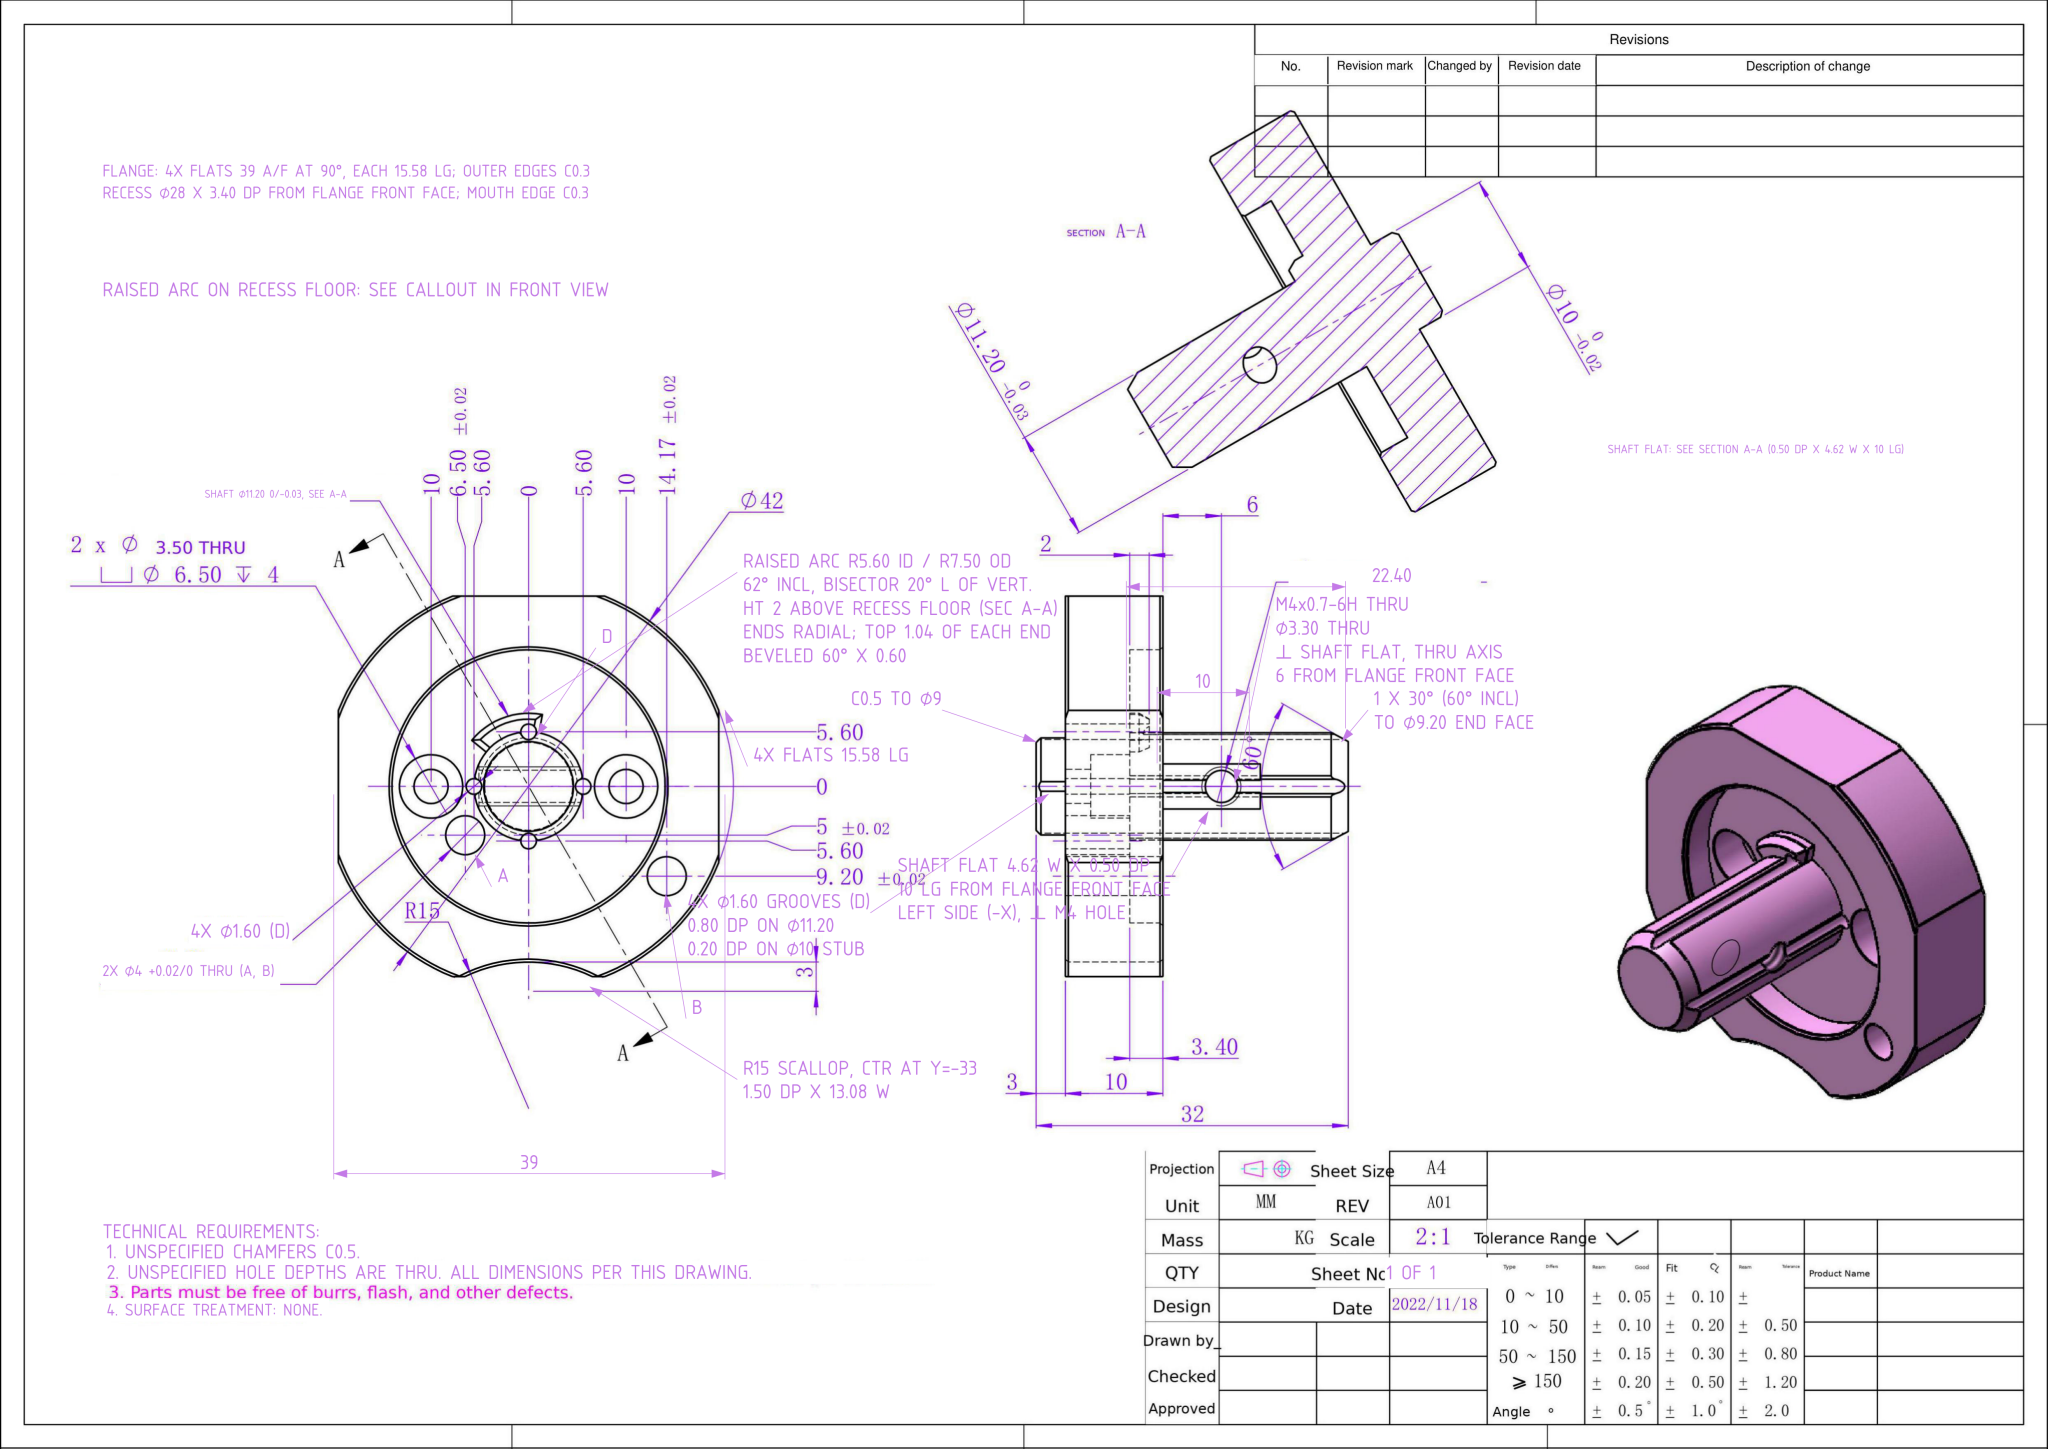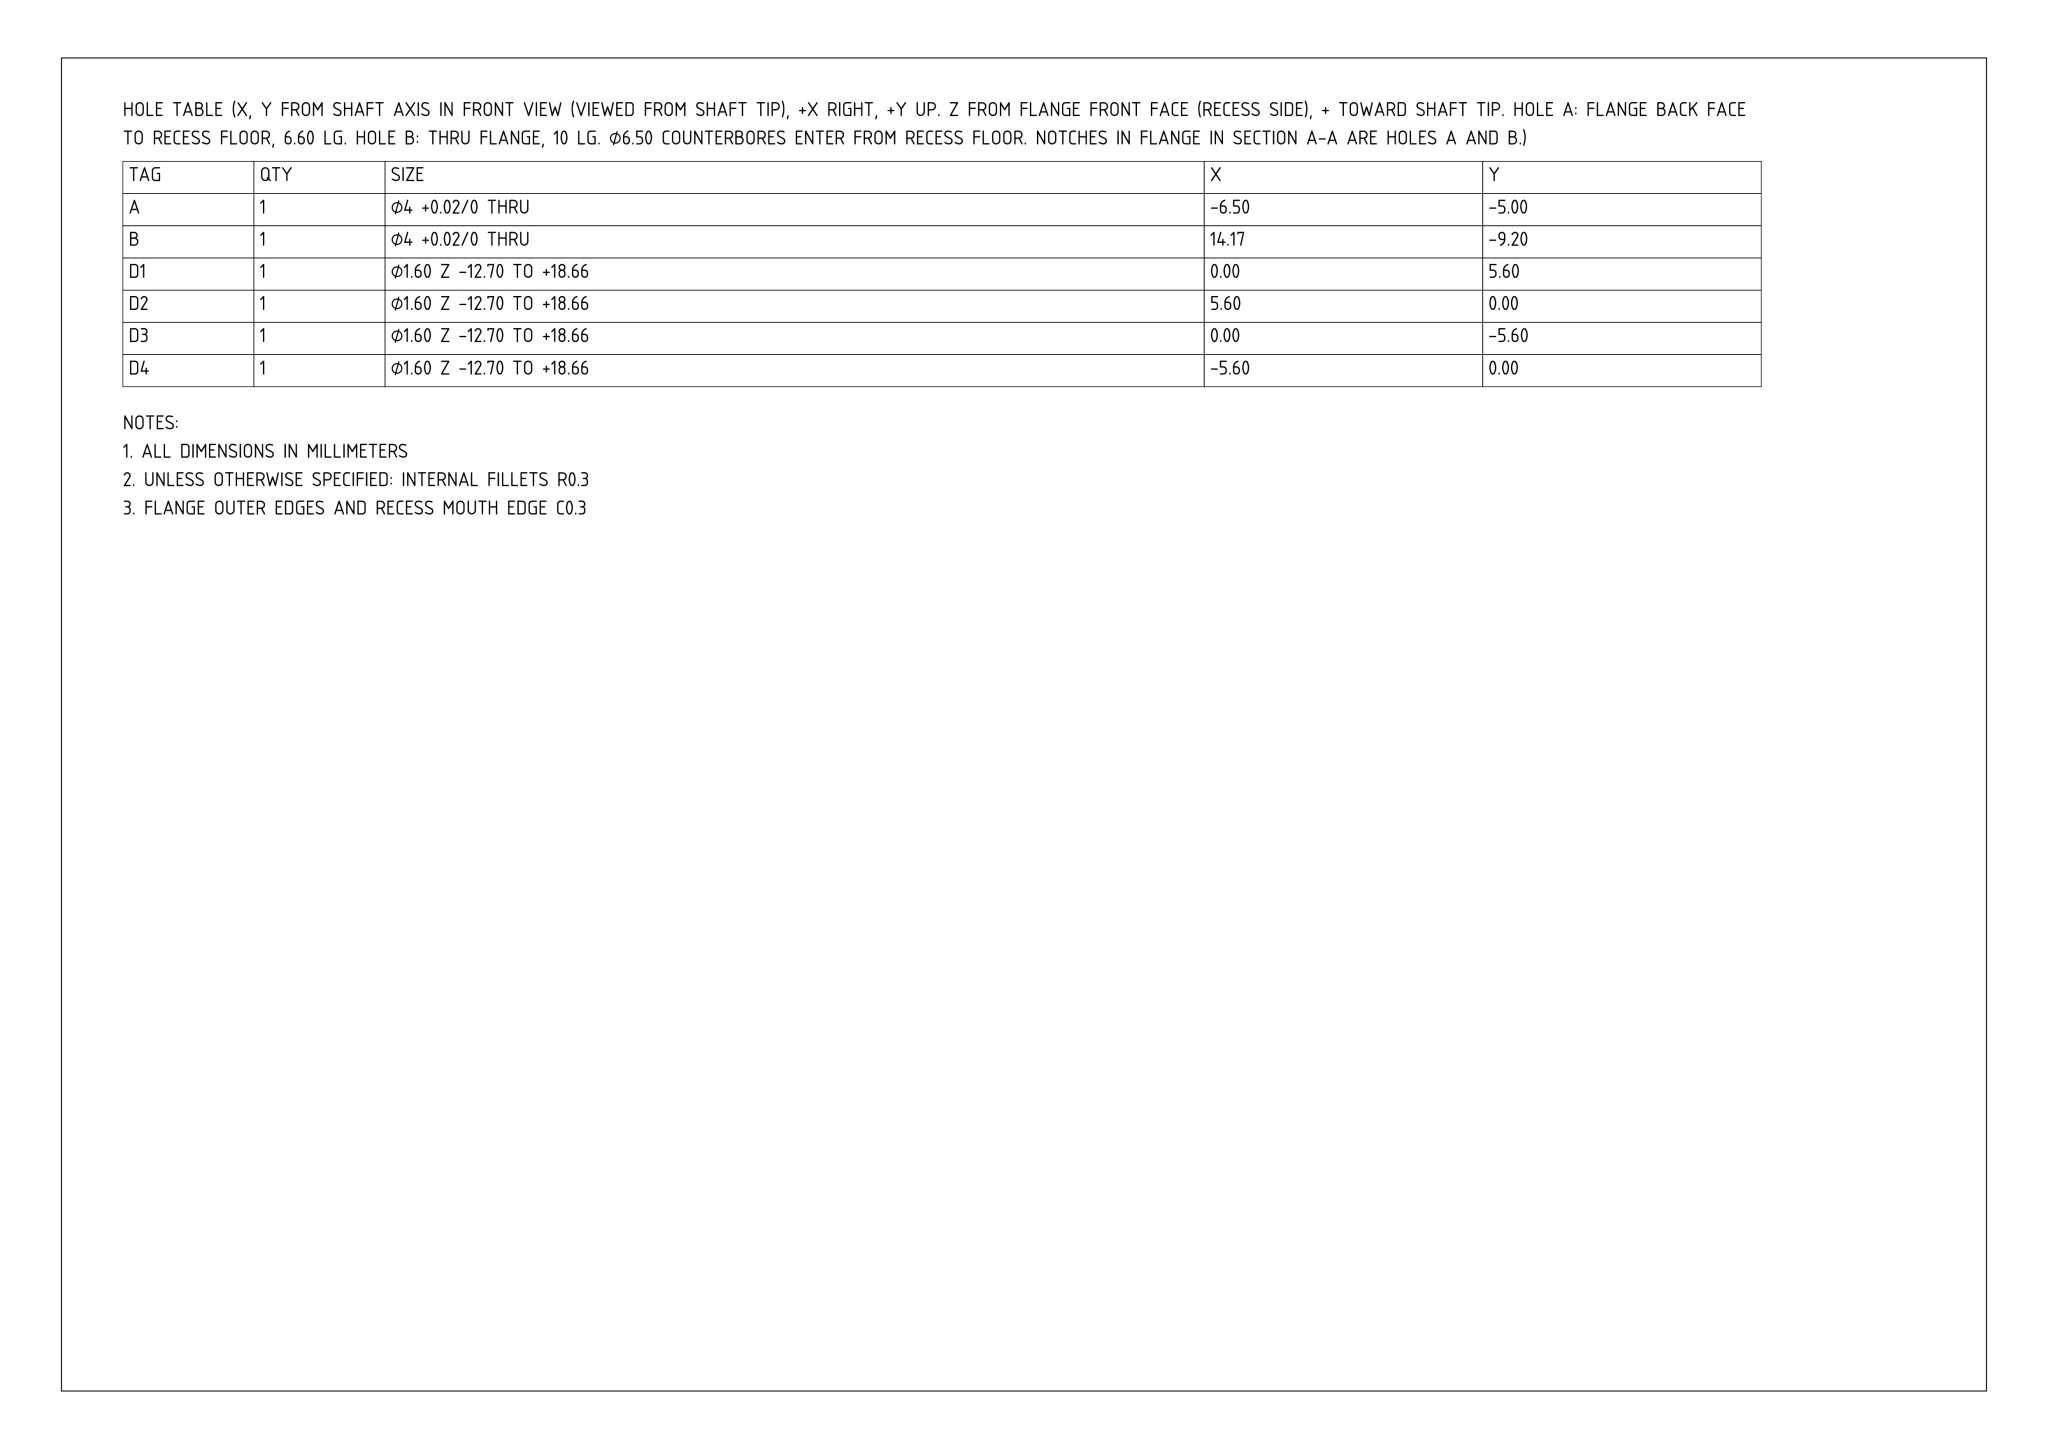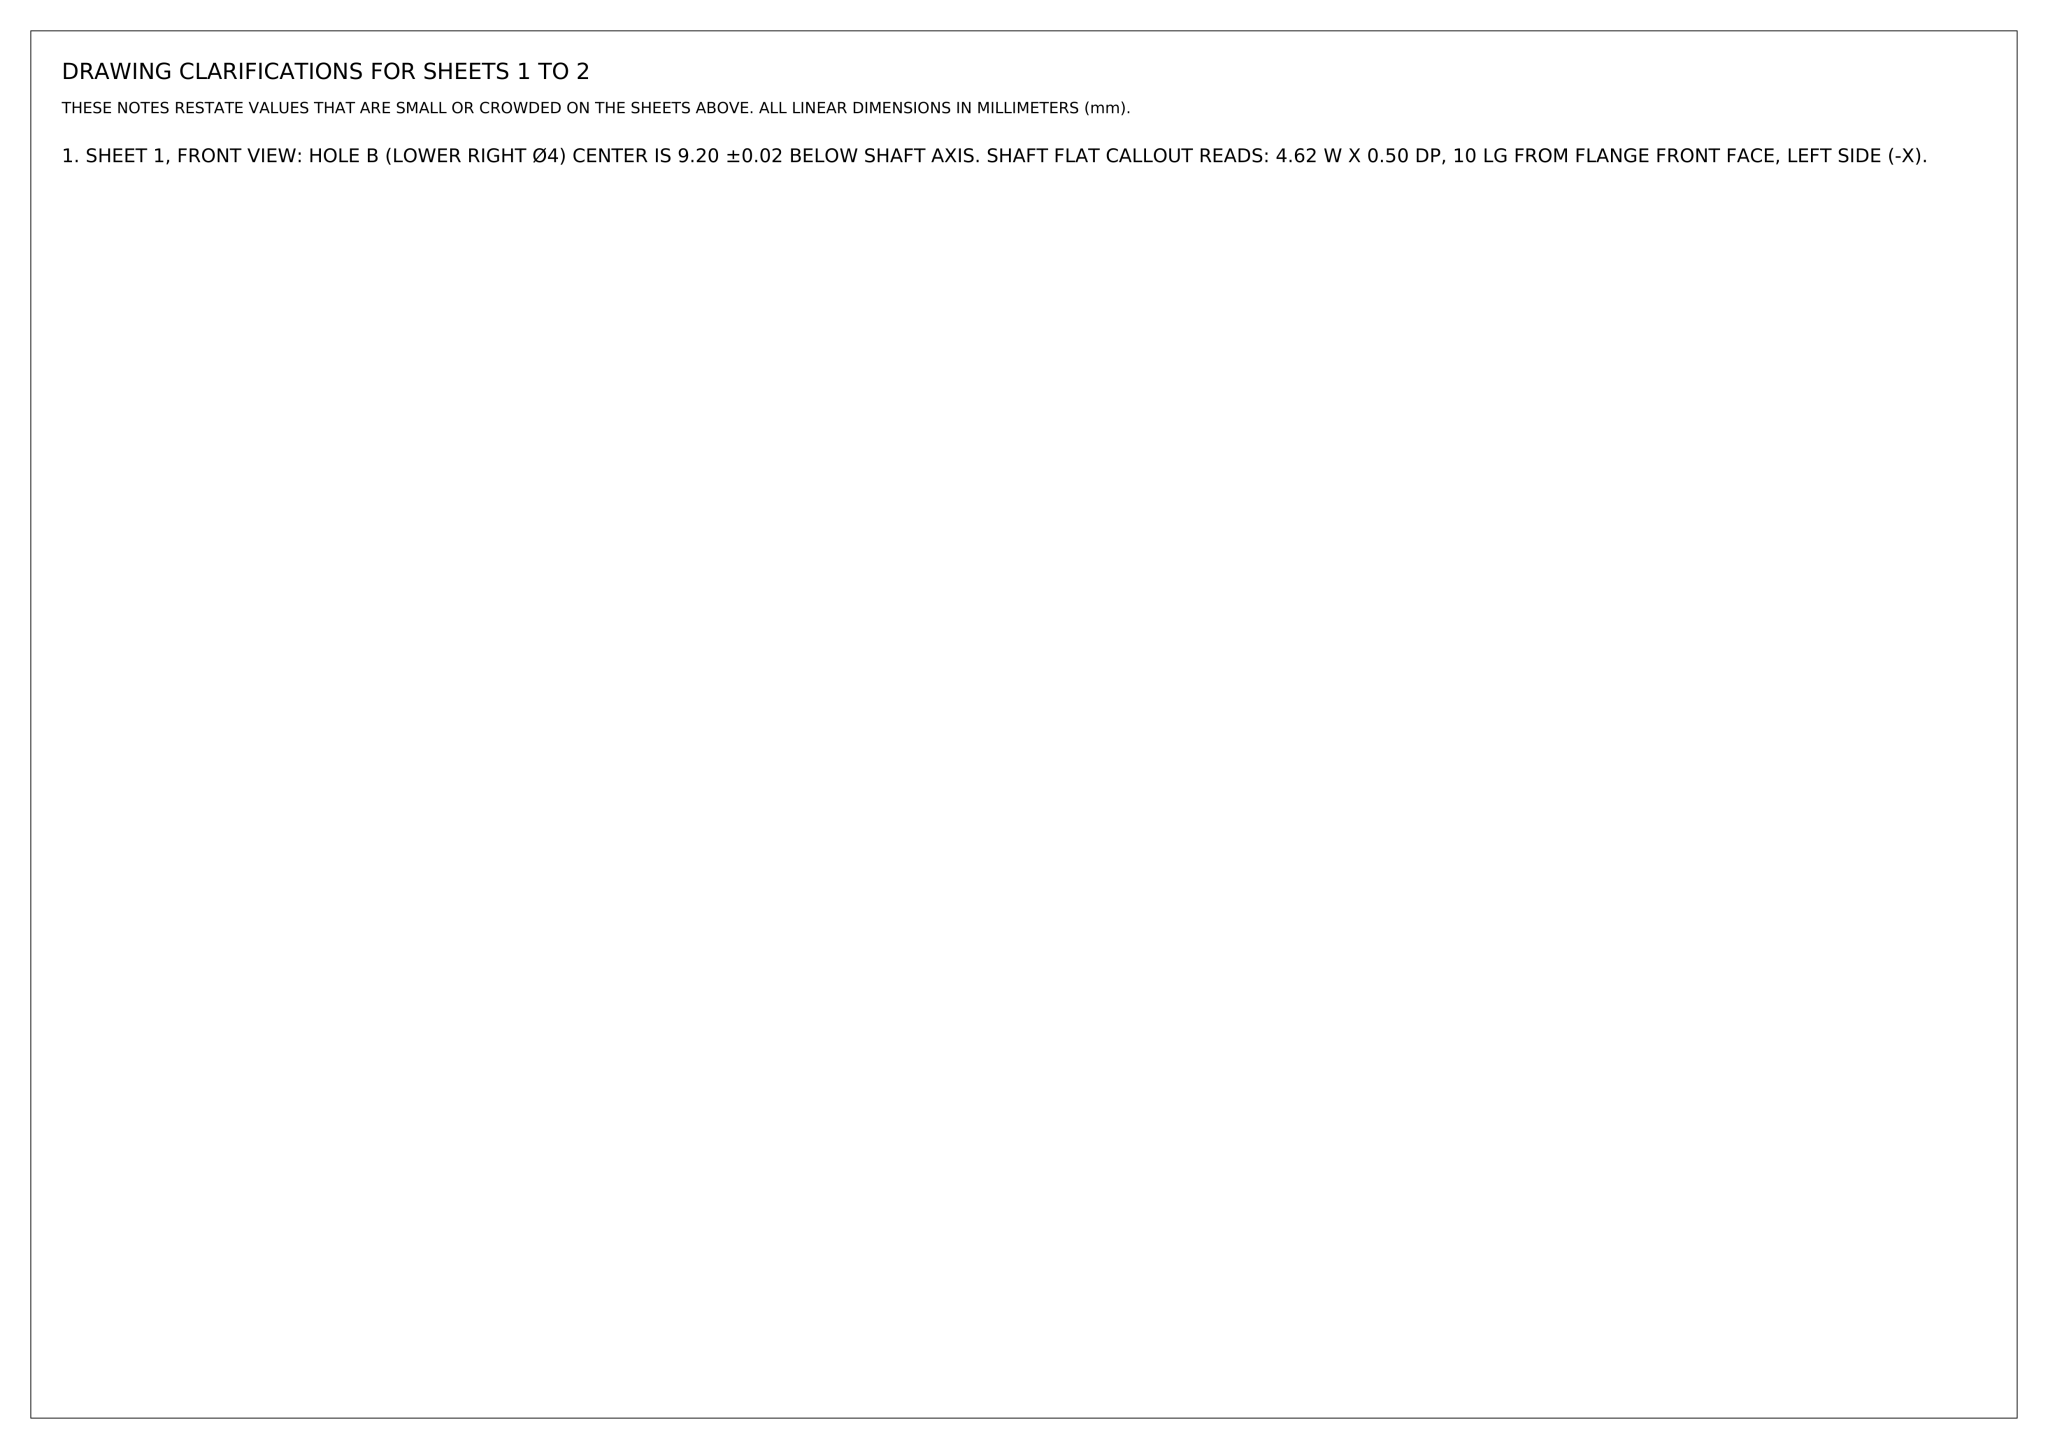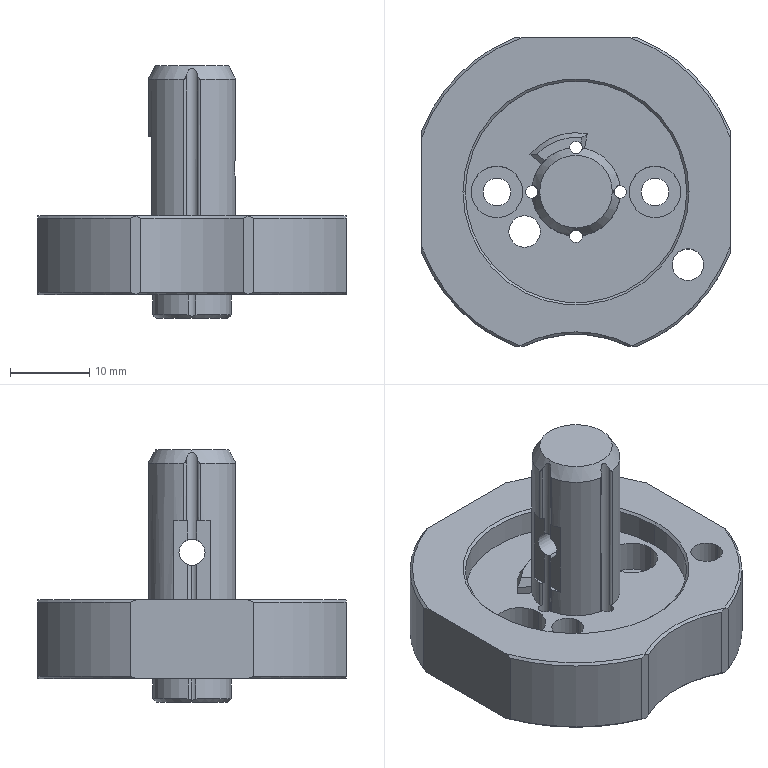Part | NX | mm | 1 solid | 97 faces | box 39 x 39 x 32 mm | volume 12662 mm3 | cylinder 57 | plane 23 | cone 17 | commonest cylinder face diameters 0.6 x16 1.6 x11 4 x4 6.5 x4 3.5 x4 11.2 x4 42 x4 10 x4